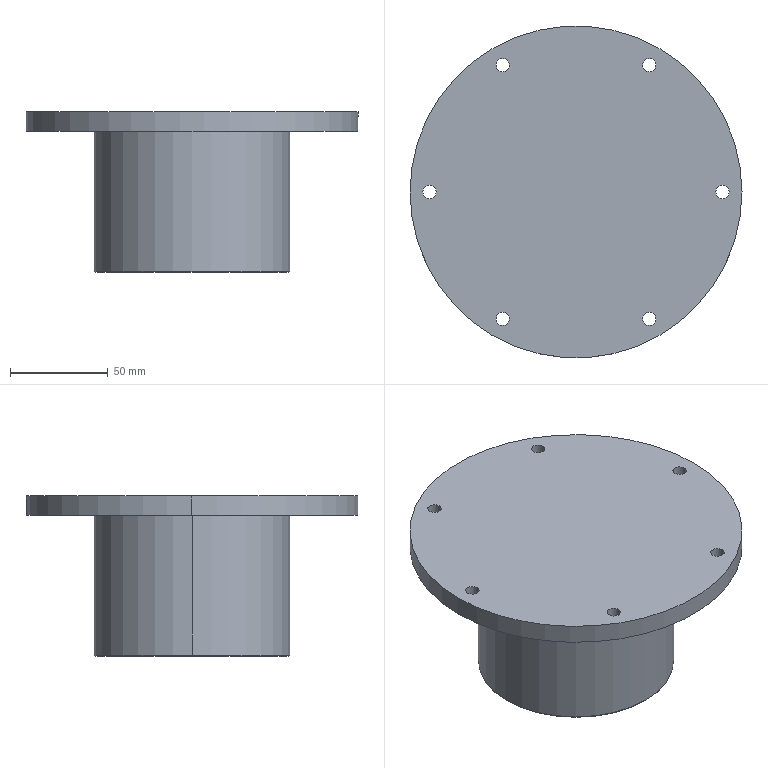Component | SolidWorks | RotatingAxis100-1 | 1 solid | 37 faces | box 170 x 170 x 82 mm | volume 789053 mm3 | cylinder 24 | cone 8 | plane 3 | torus 2 | commonest cylinder face diameters 6.8 x12 5 x8 170 x2 100 x2 | material 45#
STEP:
#1=COLOUR_RGB('',0.7922,0.8196,0.9333);
#2=FILL_AREA_STYLE_COLOUR('',#1);
#3=FILL_AREA_STYLE('',(#2));
#4=SURFACE_STYLE_FILL_AREA(#3);
#5=SURFACE_SIDE_STYLE('',(#4));
#6=SURFACE_STYLE_USAGE(.BOTH.,#5);
#7=PRESENTATION_STYLE_ASSIGNMENT((#6));
#8=CARTESIAN_POINT('',(2.019,-1.06,-50.116));
#9=VERTEX_POINT('',#8);
#10=CARTESIAN_POINT('',(-1.879,-1.06,-50.116));
#11=VERTEX_POINT('',#10);
#12=CARTESIAN_POINT('',(0.07026,-1.06,-50.116));
#13=DIRECTION('',(0.,-0.,-1.));
#14=DIRECTION('',(-1.,0.,0.));
#15=AXIS2_PLACEMENT_3D('',#12,#13,#14);
#16=CIRCLE('',#15,1.949);
#17=EDGE_CURVE('',#9,#11,#16,.T.);
#18=ORIENTED_EDGE('',*,*,#17,.F.);
#19=CARTESIAN_POINT('',(2.039,-1.06,-50.097));
#20=VERTEX_POINT('',#19);
#21=CARTESIAN_POINT('',(2.019,-1.06,-50.097));
#22=DIRECTION('',(-0.,-1.,0.));
#23=DIRECTION('',(1.,0.,0.));
#24=AXIS2_PLACEMENT_3D('',#21,#22,#23);
#25=CIRCLE('',#24,0.01969);
#26=EDGE_CURVE('',#9,#20,#25,.T.);
#27=ORIENTED_EDGE('',*,*,#26,.T.);
#28=CARTESIAN_POINT('',(-1.898,-1.06,-50.097));
#29=VERTEX_POINT('',#28);
#30=CARTESIAN_POINT('',(0.07026,-1.06,-50.097));
#31=DIRECTION('',(-0.,0.,1.));
#32=DIRECTION('',(-1.,0.,0.));
#33=AXIS2_PLACEMENT_3D('',#30,#31,#32);
#34=CIRCLE('',#33,1.969);
#35=EDGE_CURVE('',#29,#20,#34,.T.);
#36=ORIENTED_EDGE('',*,*,#35,.F.);
#37=CARTESIAN_POINT('',(-1.879,-1.06,-50.097));
#38=DIRECTION('',(0.,1.,-0.));
#39=DIRECTION('',(-1.,0.,0.));
#40=AXIS2_PLACEMENT_3D('',#37,#38,#39);
#41=CIRCLE('',#40,0.01969);
#42=EDGE_CURVE('',#11,#29,#41,.T.);
#43=ORIENTED_EDGE('',*,*,#42,.F.);
#44=EDGE_LOOP('',(#18,#27,#36,#43));
#45=FACE_OUTER_BOUND('',#44,.T.);
#46=CARTESIAN_POINT('',(0.07026,-1.06,-50.097));
#47=DIRECTION('',(-0.,0.,1.));
#48=DIRECTION('',(-1.,0.,-0.));
#49=AXIS2_PLACEMENT_3D('',#46,#47,#48);
#50=TOROIDAL_SURFACE('',#49,1.949,0.01969);
#51=ADVANCED_FACE('',(#45),#50,.T.);
#52=CARTESIAN_POINT('',(-1.142,-2.173,-49.526));
#53=VERTEX_POINT('',#52);
#54=CARTESIAN_POINT('',(-0.9449,-2.173,-49.526));
#55=VERTEX_POINT('',#54);
#56=CARTESIAN_POINT('',(-1.043,-2.173,-49.526));
#57=DIRECTION('',(0.,-0.,-1.));
#58=DIRECTION('',(1.,0.,0.));
#59=AXIS2_PLACEMENT_3D('',#56,#57,#58);
#60=CIRCLE('',#59,0.09843);
#61=EDGE_CURVE('',#53,#55,#60,.T.);
#62=ORIENTED_EDGE('',*,*,#61,.F.);
#63=CARTESIAN_POINT('',(-1.142,-2.173,-50.116));
#64=VERTEX_POINT('',#63);
#65=CARTESIAN_POINT('',(-1.142,-2.173,-50.116));
#66=DIRECTION('',(0.,-0.,-1.));
#67=VECTOR('',#66,39.37);
#68=LINE('',#65,#67);
#69=EDGE_CURVE('',#53,#64,#68,.T.);
#70=ORIENTED_EDGE('',*,*,#69,.T.);
#71=CARTESIAN_POINT('',(-0.9449,-2.173,-50.116));
#72=VERTEX_POINT('',#71);
#73=CARTESIAN_POINT('',(-1.043,-2.173,-50.116));
#74=DIRECTION('',(0.,-0.,-1.));
#75=DIRECTION('',(1.,0.,0.));
#76=AXIS2_PLACEMENT_3D('',#73,#74,#75);
#77=CIRCLE('',#76,0.09843);
#78=EDGE_CURVE('',#64,#72,#77,.T.);
#79=ORIENTED_EDGE('',*,*,#78,.T.);
#80=CARTESIAN_POINT('',(-0.9449,-2.173,-50.116));
#81=DIRECTION('',(0.,-0.,-1.));
#82=VECTOR('',#81,39.37);
#83=LINE('',#80,#82);
#84=EDGE_CURVE('',#55,#72,#83,.T.);
#85=ORIENTED_EDGE('',*,*,#84,.F.);
#86=EDGE_LOOP('',(#62,#70,#79,#85));
#87=FACE_OUTER_BOUND('',#86,.T.);
#88=CARTESIAN_POINT('',(-1.043,-2.173,-50.116));
#89=DIRECTION('',(0.,-0.,-1.));
#90=DIRECTION('',(1.,0.,0.));
#91=AXIS2_PLACEMENT_3D('',#88,#89,#90);
#92=CYLINDRICAL_SURFACE('',#91,0.09843);
#93=ADVANCED_FACE('',(#87),#92,.F.);
#94=CARTESIAN_POINT('',(-1.043,-2.173,-49.467));
#95=VERTEX_POINT('',#94);
#96=CARTESIAN_POINT('',(-0.9449,-2.173,-49.526));
#97=DIRECTION('',(0.8572,-0.,-0.515));
#98=VECTOR('',#97,39.37);
#99=LINE('',#96,#98);
#100=EDGE_CURVE('',#95,#55,#99,.T.);
#101=ORIENTED_EDGE('',*,*,#100,.F.);
#102=CARTESIAN_POINT('',(-1.142,-2.173,-49.526));
#103=DIRECTION('',(-0.8572,0.,-0.515));
#104=VECTOR('',#103,39.37);
#105=LINE('',#102,#104);
#106=EDGE_CURVE('',#95,#53,#105,.T.);
#107=ORIENTED_EDGE('',*,*,#106,.T.);
#108=ORIENTED_EDGE('',*,*,#61,.T.);
#109=EDGE_LOOP('',(#101,#107,#108));
#110=FACE_OUTER_BOUND('',#109,.T.);
#111=CARTESIAN_POINT('',(-1.043,-2.173,-49.526));
#112=DIRECTION('',(0.,-0.,-1.));
#113=DIRECTION('',(1.,0.,0.));
#114=AXIS2_PLACEMENT_3D('',#111,#112,#113);
#115=CONICAL_SURFACE('',#114,0.09843,1.03);
#116=ADVANCED_FACE('',(#110),#115,.F.);
#117=CARTESIAN_POINT('',(1.085,-2.173,-49.526));
#118=VERTEX_POINT('',#117);
#119=CARTESIAN_POINT('',(1.282,-2.173,-49.526));
#120=VERTEX_POINT('',#119);
#121=CARTESIAN_POINT('',(1.184,-2.173,-49.526));
#122=DIRECTION('',(0.,-0.,-1.));
#123=DIRECTION('',(1.,0.,0.));
#124=AXIS2_PLACEMENT_3D('',#121,#122,#123);
#125=CIRCLE('',#124,0.09843);
#126=EDGE_CURVE('',#118,#120,#125,.T.);
#127=ORIENTED_EDGE('',*,*,#126,.F.);
#128=CARTESIAN_POINT('',(1.085,-2.173,-50.116));
#129=VERTEX_POINT('',#128);
#130=CARTESIAN_POINT('',(1.085,-2.173,-50.116));
#131=DIRECTION('',(0.,-0.,-1.));
#132=VECTOR('',#131,39.37);
#133=LINE('',#130,#132);
#134=EDGE_CURVE('',#118,#129,#133,.T.);
#135=ORIENTED_EDGE('',*,*,#134,.T.);
#136=CARTESIAN_POINT('',(1.282,-2.173,-50.116));
#137=VERTEX_POINT('',#136);
#138=CARTESIAN_POINT('',(1.184,-2.173,-50.116));
#139=DIRECTION('',(0.,-0.,-1.));
#140=DIRECTION('',(1.,0.,0.));
#141=AXIS2_PLACEMENT_3D('',#138,#139,#140);
#142=CIRCLE('',#141,0.09843);
#143=EDGE_CURVE('',#129,#137,#142,.T.);
#144=ORIENTED_EDGE('',*,*,#143,.T.);
#145=CARTESIAN_POINT('',(1.282,-2.173,-50.116));
#146=DIRECTION('',(0.,-0.,-1.));
#147=VECTOR('',#146,39.37);
#148=LINE('',#145,#147);
#149=EDGE_CURVE('',#120,#137,#148,.T.);
#150=ORIENTED_EDGE('',*,*,#149,.F.);
#151=EDGE_LOOP('',(#127,#135,#144,#150));
#152=FACE_OUTER_BOUND('',#151,.T.);
#153=CARTESIAN_POINT('',(1.184,-2.173,-50.116));
#154=DIRECTION('',(0.,-0.,-1.));
#155=DIRECTION('',(1.,0.,0.));
#156=AXIS2_PLACEMENT_3D('',#153,#154,#155);
#157=CYLINDRICAL_SURFACE('',#156,0.09843);
#158=ADVANCED_FACE('',(#152),#157,.F.);
#159=CARTESIAN_POINT('',(1.184,-2.173,-49.467));
#160=VERTEX_POINT('',#159);
#161=CARTESIAN_POINT('',(1.282,-2.173,-49.526));
#162=DIRECTION('',(0.8572,-0.,-0.515));
#163=VECTOR('',#162,39.37);
#164=LINE('',#161,#163);
#165=EDGE_CURVE('',#160,#120,#164,.T.);
#166=ORIENTED_EDGE('',*,*,#165,.F.);
#167=CARTESIAN_POINT('',(1.085,-2.173,-49.526));
#168=DIRECTION('',(-0.8572,0.,-0.515));
#169=VECTOR('',#168,39.37);
#170=LINE('',#167,#169);
#171=EDGE_CURVE('',#160,#118,#170,.T.);
#172=ORIENTED_EDGE('',*,*,#171,.T.);
#173=ORIENTED_EDGE('',*,*,#126,.T.);
#174=EDGE_LOOP('',(#166,#172,#173));
#175=FACE_OUTER_BOUND('',#174,.T.);
#176=CARTESIAN_POINT('',(1.184,-2.173,-49.526));
#177=DIRECTION('',(0.,-0.,-1.));
#178=DIRECTION('',(1.,0.,0.));
#179=AXIS2_PLACEMENT_3D('',#176,#177,#178);
#180=CONICAL_SURFACE('',#179,0.09843,1.03);
#181=ADVANCED_FACE('',(#175),#180,.F.);
#182=CARTESIAN_POINT('',(1.085,0.05383,-49.526));
#183=VERTEX_POINT('',#182);
#184=CARTESIAN_POINT('',(1.282,0.05383,-49.526));
#185=VERTEX_POINT('',#184);
#186=CARTESIAN_POINT('',(1.184,0.05383,-49.526));
#187=DIRECTION('',(0.,-0.,-1.));
#188=DIRECTION('',(1.,-0.,0.));
#189=AXIS2_PLACEMENT_3D('',#186,#187,#188);
#190=CIRCLE('',#189,0.09843);
#191=EDGE_CURVE('',#183,#185,#190,.T.);
#192=ORIENTED_EDGE('',*,*,#191,.F.);
#193=CARTESIAN_POINT('',(1.085,0.05383,-50.116));
#194=VERTEX_POINT('',#193);
#195=CARTESIAN_POINT('',(1.085,0.05383,-50.116));
#196=DIRECTION('',(0.,-0.,-1.));
#197=VECTOR('',#196,39.37);
#198=LINE('',#195,#197);
#199=EDGE_CURVE('',#183,#194,#198,.T.);
#200=ORIENTED_EDGE('',*,*,#199,.T.);
#201=CARTESIAN_POINT('',(1.282,0.05383,-50.116));
#202=VERTEX_POINT('',#201);
#203=CARTESIAN_POINT('',(1.184,0.05383,-50.116));
#204=DIRECTION('',(0.,-0.,-1.));
#205=DIRECTION('',(1.,-0.,0.));
#206=AXIS2_PLACEMENT_3D('',#203,#204,#205);
#207=CIRCLE('',#206,0.09843);
#208=EDGE_CURVE('',#194,#202,#207,.T.);
#209=ORIENTED_EDGE('',*,*,#208,.T.);
#210=CARTESIAN_POINT('',(1.282,0.05383,-50.116));
#211=DIRECTION('',(0.,-0.,-1.));
#212=VECTOR('',#211,39.37);
#213=LINE('',#210,#212);
#214=EDGE_CURVE('',#185,#202,#213,.T.);
#215=ORIENTED_EDGE('',*,*,#214,.F.);
#216=EDGE_LOOP('',(#192,#200,#209,#215));
#217=FACE_OUTER_BOUND('',#216,.T.);
#218=CARTESIAN_POINT('',(1.184,0.05383,-50.116));
#219=DIRECTION('',(0.,-0.,-1.));
#220=DIRECTION('',(1.,-0.,0.));
#221=AXIS2_PLACEMENT_3D('',#218,#219,#220);
#222=CYLINDRICAL_SURFACE('',#221,0.09843);
#223=ADVANCED_FACE('',(#217),#222,.F.);
#224=CARTESIAN_POINT('',(1.184,0.05383,-49.467));
#225=VERTEX_POINT('',#224);
#226=CARTESIAN_POINT('',(1.282,0.05383,-49.526));
#227=DIRECTION('',(0.8572,-0.,-0.515));
#228=VECTOR('',#227,39.37);
#229=LINE('',#226,#228);
#230=EDGE_CURVE('',#225,#185,#229,.T.);
#231=ORIENTED_EDGE('',*,*,#230,.F.);
#232=CARTESIAN_POINT('',(1.085,0.05383,-49.526));
#233=DIRECTION('',(-0.8572,0.,-0.515));
#234=VECTOR('',#233,39.37);
#235=LINE('',#232,#234);
#236=EDGE_CURVE('',#225,#183,#235,.T.);
#237=ORIENTED_EDGE('',*,*,#236,.T.);
#238=ORIENTED_EDGE('',*,*,#191,.T.);
#239=EDGE_LOOP('',(#231,#237,#238));
#240=FACE_OUTER_BOUND('',#239,.T.);
#241=CARTESIAN_POINT('',(1.184,0.05383,-49.526));
#242=DIRECTION('',(0.,-0.,-1.));
#243=DIRECTION('',(1.,-0.,0.));
#244=AXIS2_PLACEMENT_3D('',#241,#242,#243);
#245=CONICAL_SURFACE('',#244,0.09843,1.03);
#246=ADVANCED_FACE('',(#240),#245,.F.);
#247=CARTESIAN_POINT('',(-1.142,0.05383,-49.526));
#248=VERTEX_POINT('',#247);
#249=CARTESIAN_POINT('',(-0.9449,0.05383,-49.526));
#250=VERTEX_POINT('',#249);
#251=CARTESIAN_POINT('',(-1.043,0.05383,-49.526));
#252=DIRECTION('',(0.,-0.,-1.));
#253=DIRECTION('',(1.,-0.,0.));
#254=AXIS2_PLACEMENT_3D('',#251,#252,#253);
#255=CIRCLE('',#254,0.09843);
#256=EDGE_CURVE('',#248,#250,#255,.T.);
#257=ORIENTED_EDGE('',*,*,#256,.F.);
#258=CARTESIAN_POINT('',(-1.142,0.05383,-50.116));
#259=VERTEX_POINT('',#258);
#260=CARTESIAN_POINT('',(-1.142,0.05383,-50.116));
#261=DIRECTION('',(0.,-0.,-1.));
#262=VECTOR('',#261,39.37);
#263=LINE('',#260,#262);
#264=EDGE_CURVE('',#248,#259,#263,.T.);
#265=ORIENTED_EDGE('',*,*,#264,.T.);
#266=CARTESIAN_POINT('',(-0.9449,0.05383,-50.116));
#267=VERTEX_POINT('',#266);
#268=CARTESIAN_POINT('',(-1.043,0.05383,-50.116));
#269=DIRECTION('',(0.,-0.,-1.));
#270=DIRECTION('',(1.,-0.,0.));
#271=AXIS2_PLACEMENT_3D('',#268,#269,#270);
#272=CIRCLE('',#271,0.09843);
#273=EDGE_CURVE('',#259,#267,#272,.T.);
#274=ORIENTED_EDGE('',*,*,#273,.T.);
#275=CARTESIAN_POINT('',(-0.9449,0.05383,-50.116));
#276=DIRECTION('',(0.,-0.,-1.));
#277=VECTOR('',#276,39.37);
#278=LINE('',#275,#277);
#279=EDGE_CURVE('',#250,#267,#278,.T.);
#280=ORIENTED_EDGE('',*,*,#279,.F.);
#281=EDGE_LOOP('',(#257,#265,#274,#280));
#282=FACE_OUTER_BOUND('',#281,.T.);
#283=CARTESIAN_POINT('',(-1.043,0.05383,-50.116));
#284=DIRECTION('',(0.,-0.,-1.));
#285=DIRECTION('',(1.,-0.,0.));
#286=AXIS2_PLACEMENT_3D('',#283,#284,#285);
#287=CYLINDRICAL_SURFACE('',#286,0.09843);
#288=ADVANCED_FACE('',(#282),#287,.F.);
#289=CARTESIAN_POINT('',(-1.043,0.05383,-49.467));
#290=VERTEX_POINT('',#289);
#291=CARTESIAN_POINT('',(-0.9449,0.05383,-49.526));
#292=DIRECTION('',(0.8572,-0.,-0.515));
#293=VECTOR('',#292,39.37);
#294=LINE('',#291,#293);
#295=EDGE_CURVE('',#290,#250,#294,.T.);
#296=ORIENTED_EDGE('',*,*,#295,.F.);
#297=CARTESIAN_POINT('',(-1.142,0.05383,-49.526));
#298=DIRECTION('',(-0.8572,0.,-0.515));
#299=VECTOR('',#298,39.37);
#300=LINE('',#297,#299);
#301=EDGE_CURVE('',#290,#248,#300,.T.);
#302=ORIENTED_EDGE('',*,*,#301,.T.);
#303=ORIENTED_EDGE('',*,*,#256,.T.);
#304=EDGE_LOOP('',(#296,#302,#303));
#305=FACE_OUTER_BOUND('',#304,.T.);
#306=CARTESIAN_POINT('',(-1.043,0.05383,-49.526));
#307=DIRECTION('',(0.,-0.,-1.));
#308=DIRECTION('',(1.,-0.,0.));
#309=AXIS2_PLACEMENT_3D('',#306,#307,#308);
#310=CONICAL_SURFACE('',#309,0.09843,1.03);
#311=ADVANCED_FACE('',(#305),#310,.F.);
#312=CARTESIAN_POINT('',(1.681,-3.617,-47.282));
#313=VERTEX_POINT('',#312);
#314=CARTESIAN_POINT('',(1.413,-3.617,-47.282));
#315=VERTEX_POINT('',#314);
#316=CARTESIAN_POINT('',(1.547,-3.617,-47.282));
#317=DIRECTION('',(-0.,0.,1.));
#318=DIRECTION('',(-1.,0.,0.));
#319=AXIS2_PLACEMENT_3D('',#316,#317,#318);
#320=CIRCLE('',#319,0.1339);
#321=EDGE_CURVE('',#313,#315,#320,.T.);
#322=ORIENTED_EDGE('',*,*,#321,.F.);
#323=CARTESIAN_POINT('',(1.681,-3.617,-46.888));
#324=VERTEX_POINT('',#323);
#325=CARTESIAN_POINT('',(1.681,-3.617,-46.888));
#326=DIRECTION('',(-0.,0.,1.));
#327=VECTOR('',#326,39.37);
#328=LINE('',#325,#327);
#329=EDGE_CURVE('',#313,#324,#328,.T.);
#330=ORIENTED_EDGE('',*,*,#329,.T.);
#331=CARTESIAN_POINT('',(1.413,-3.617,-46.888));
#332=VERTEX_POINT('',#331);
#333=CARTESIAN_POINT('',(1.547,-3.617,-46.888));
#334=DIRECTION('',(-0.,0.,1.));
#335=DIRECTION('',(-1.,0.,0.));
#336=AXIS2_PLACEMENT_3D('',#333,#334,#335);
#337=CIRCLE('',#336,0.1339);
#338=EDGE_CURVE('',#324,#332,#337,.T.);
#339=ORIENTED_EDGE('',*,*,#338,.T.);
#340=CARTESIAN_POINT('',(1.413,-3.617,-46.888));
#341=DIRECTION('',(-0.,0.,1.));
#342=VECTOR('',#341,39.37);
#343=LINE('',#340,#342);
#344=EDGE_CURVE('',#315,#332,#343,.T.);
#345=ORIENTED_EDGE('',*,*,#344,.F.);
#346=EDGE_LOOP('',(#322,#330,#339,#345));
#347=FACE_OUTER_BOUND('',#346,.T.);
#348=CARTESIAN_POINT('',(1.547,-3.617,-46.888));
#349=DIRECTION('',(-0.,0.,1.));
#350=DIRECTION('',(-1.,0.,0.));
#351=AXIS2_PLACEMENT_3D('',#348,#349,#350);
#352=CYLINDRICAL_SURFACE('',#351,0.1339);
#353=ADVANCED_FACE('',(#347),#352,.F.);
#354=CARTESIAN_POINT('',(-1.272,-3.617,-47.282));
#355=VERTEX_POINT('',#354);
#356=CARTESIAN_POINT('',(-1.54,-3.617,-47.282));
#357=VERTEX_POINT('',#356);
#358=CARTESIAN_POINT('',(-1.406,-3.617,-47.282));
#359=DIRECTION('',(-0.,0.,1.));
#360=DIRECTION('',(-1.,0.,0.));
#361=AXIS2_PLACEMENT_3D('',#358,#359,#360);
#362=CIRCLE('',#361,0.1339);
#363=EDGE_CURVE('',#355,#357,#362,.T.);
#364=ORIENTED_EDGE('',*,*,#363,.F.);
#365=CARTESIAN_POINT('',(-1.272,-3.617,-46.888));
#366=VERTEX_POINT('',#365);
#367=CARTESIAN_POINT('',(-1.272,-3.617,-46.888));
#368=DIRECTION('',(-0.,0.,1.));
#369=VECTOR('',#368,39.37);
#370=LINE('',#367,#369);
#371=EDGE_CURVE('',#355,#366,#370,.T.);
#372=ORIENTED_EDGE('',*,*,#371,.T.);
#373=CARTESIAN_POINT('',(-1.54,-3.617,-46.888));
#374=VERTEX_POINT('',#373);
#375=CARTESIAN_POINT('',(-1.406,-3.617,-46.888));
#376=DIRECTION('',(-0.,0.,1.));
#377=DIRECTION('',(-1.,0.,0.));
#378=AXIS2_PLACEMENT_3D('',#375,#376,#377);
#379=CIRCLE('',#378,0.1339);
#380=EDGE_CURVE('',#366,#374,#379,.T.);
#381=ORIENTED_EDGE('',*,*,#380,.T.);
#382=CARTESIAN_POINT('',(-1.54,-3.617,-46.888));
#383=DIRECTION('',(-0.,0.,1.));
#384=VECTOR('',#383,39.37);
#385=LINE('',#382,#384);
#386=EDGE_CURVE('',#357,#374,#385,.T.);
#387=ORIENTED_EDGE('',*,*,#386,.F.);
#388=EDGE_LOOP('',(#364,#372,#381,#387));
#389=FACE_OUTER_BOUND('',#388,.T.);
#390=CARTESIAN_POINT('',(-1.406,-3.617,-46.888));
#391=DIRECTION('',(-0.,0.,1.));
#392=DIRECTION('',(-1.,0.,0.));
#393=AXIS2_PLACEMENT_3D('',#390,#391,#392);
#394=CYLINDRICAL_SURFACE('',#393,0.1339);
#395=ADVANCED_FACE('',(#389),#394,.F.);
#396=CARTESIAN_POINT('',(-2.749,-1.06,-47.282));
#397=VERTEX_POINT('',#396);
#398=CARTESIAN_POINT('',(-3.016,-1.06,-47.282));
#399=VERTEX_POINT('',#398);
#400=CARTESIAN_POINT('',(-2.882,-1.06,-47.282));
#401=DIRECTION('',(-0.,0.,1.));
#402=DIRECTION('',(-1.,0.,0.));
#403=AXIS2_PLACEMENT_3D('',#400,#401,#402);
#404=CIRCLE('',#403,0.1339);
#405=EDGE_CURVE('',#397,#399,#404,.T.);
#406=ORIENTED_EDGE('',*,*,#405,.F.);
#407=CARTESIAN_POINT('',(-2.749,-1.06,-46.888));
#408=VERTEX_POINT('',#407);
#409=CARTESIAN_POINT('',(-2.749,-1.06,-46.888));
#410=DIRECTION('',(-0.,0.,1.));
#411=VECTOR('',#410,39.37);
#412=LINE('',#409,#411);
#413=EDGE_CURVE('',#397,#408,#412,.T.);
#414=ORIENTED_EDGE('',*,*,#413,.T.);
#415=CARTESIAN_POINT('',(-3.016,-1.06,-46.888));
#416=VERTEX_POINT('',#415);
#417=CARTESIAN_POINT('',(-2.882,-1.06,-46.888));
#418=DIRECTION('',(-0.,0.,1.));
#419=DIRECTION('',(-1.,0.,0.));
#420=AXIS2_PLACEMENT_3D('',#417,#418,#419);
#421=CIRCLE('',#420,0.1339);
#422=EDGE_CURVE('',#408,#416,#421,.T.);
#423=ORIENTED_EDGE('',*,*,#422,.T.);
#424=CARTESIAN_POINT('',(-3.016,-1.06,-46.888));
#425=DIRECTION('',(-0.,0.,1.));
#426=VECTOR('',#425,39.37);
#427=LINE('',#424,#426);
#428=EDGE_CURVE('',#399,#416,#427,.T.);
#429=ORIENTED_EDGE('',*,*,#428,.F.);
#430=EDGE_LOOP('',(#406,#414,#423,#429));
#431=FACE_OUTER_BOUND('',#430,.T.);
#432=CARTESIAN_POINT('',(-2.882,-1.06,-46.888));
#433=DIRECTION('',(-0.,0.,1.));
#434=DIRECTION('',(-1.,0.,0.));
#435=AXIS2_PLACEMENT_3D('',#432,#433,#434);
#436=CYLINDRICAL_SURFACE('',#435,0.1339);
#437=ADVANCED_FACE('',(#431),#436,.F.);
#438=CARTESIAN_POINT('',(-1.272,1.497,-47.282));
#439=VERTEX_POINT('',#438);
#440=CARTESIAN_POINT('',(-1.54,1.497,-47.282));
#441=VERTEX_POINT('',#440);
#442=CARTESIAN_POINT('',(-1.406,1.497,-47.282));
#443=DIRECTION('',(-0.,0.,1.));
#444=DIRECTION('',(-1.,0.,0.));
#445=AXIS2_PLACEMENT_3D('',#442,#443,#444);
#446=CIRCLE('',#445,0.1339);
#447=EDGE_CURVE('',#439,#441,#446,.T.);
#448=ORIENTED_EDGE('',*,*,#447,.F.);
#449=CARTESIAN_POINT('',(-1.272,1.497,-46.888));
#450=VERTEX_POINT('',#449);
#451=CARTESIAN_POINT('',(-1.272,1.497,-46.888));
#452=DIRECTION('',(-0.,0.,1.));
#453=VECTOR('',#452,39.37);
#454=LINE('',#451,#453);
#455=EDGE_CURVE('',#439,#450,#454,.T.);
#456=ORIENTED_EDGE('',*,*,#455,.T.);
#457=CARTESIAN_POINT('',(-1.54,1.497,-46.888));
#458=VERTEX_POINT('',#457);
#459=CARTESIAN_POINT('',(-1.406,1.497,-46.888));
#460=DIRECTION('',(-0.,0.,1.));
#461=DIRECTION('',(-1.,0.,0.));
#462=AXIS2_PLACEMENT_3D('',#459,#460,#461);
#463=CIRCLE('',#462,0.1339);
#464=EDGE_CURVE('',#450,#458,#463,.T.);
#465=ORIENTED_EDGE('',*,*,#464,.T.);
#466=CARTESIAN_POINT('',(-1.54,1.497,-46.888));
#467=DIRECTION('',(-0.,0.,1.));
#468=VECTOR('',#467,39.37);
#469=LINE('',#466,#468);
#470=EDGE_CURVE('',#441,#458,#469,.T.);
#471=ORIENTED_EDGE('',*,*,#470,.F.);
#472=EDGE_LOOP('',(#448,#456,#465,#471));
#473=FACE_OUTER_BOUND('',#472,.T.);
#474=CARTESIAN_POINT('',(-1.406,1.497,-46.888));
#475=DIRECTION('',(-0.,0.,1.));
#476=DIRECTION('',(-1.,0.,0.));
#477=AXIS2_PLACEMENT_3D('',#474,#475,#476);
#478=CYLINDRICAL_SURFACE('',#477,0.1339);
#479=ADVANCED_FACE('',(#473),#478,.F.);
#480=CARTESIAN_POINT('',(1.681,1.497,-47.282));
#481=VERTEX_POINT('',#480);
#482=CARTESIAN_POINT('',(1.413,1.497,-47.282));
#483=VERTEX_POINT('',#482);
#484=CARTESIAN_POINT('',(1.547,1.497,-47.282));
#485=DIRECTION('',(-0.,0.,1.));
#486=DIRECTION('',(-1.,0.,0.));
#487=AXIS2_PLACEMENT_3D('',#484,#485,#486);
#488=CIRCLE('',#487,0.1339);
#489=EDGE_CURVE('',#481,#483,#488,.T.);
#490=ORIENTED_EDGE('',*,*,#489,.F.);
#491=CARTESIAN_POINT('',(1.681,1.497,-46.888));
#492=VERTEX_POINT('',#491);
#493=CARTESIAN_POINT('',(1.681,1.497,-46.888));
#494=DIRECTION('',(-0.,0.,1.));
#495=VECTOR('',#494,39.37);
#496=LINE('',#493,#495);
#497=EDGE_CURVE('',#481,#492,#496,.T.);
#498=ORIENTED_EDGE('',*,*,#497,.T.);
#499=CARTESIAN_POINT('',(1.413,1.497,-46.888));
#500=VERTEX_POINT('',#499);
#501=CARTESIAN_POINT('',(1.547,1.497,-46.888));
#502=DIRECTION('',(-0.,0.,1.));
#503=DIRECTION('',(-1.,0.,0.));
#504=AXIS2_PLACEMENT_3D('',#501,#502,#503);
#505=CIRCLE('',#504,0.1339);
#506=EDGE_CURVE('',#492,#500,#505,.T.);
#507=ORIENTED_EDGE('',*,*,#506,.T.);
#508=CARTESIAN_POINT('',(1.413,1.497,-46.888));
#509=DIRECTION('',(-0.,0.,1.));
#510=VECTOR('',#509,39.37);
#511=LINE('',#508,#510);
#512=EDGE_CURVE('',#483,#500,#511,.T.);
#513=ORIENTED_EDGE('',*,*,#512,.F.);
#514=EDGE_LOOP('',(#490,#498,#507,#513));
#515=FACE_OUTER_BOUND('',#514,.T.);
#516=CARTESIAN_POINT('',(1.547,1.497,-46.888));
#517=DIRECTION('',(-0.,0.,1.));
#518=DIRECTION('',(-1.,0.,0.));
#519=AXIS2_PLACEMENT_3D('',#516,#517,#518);
#520=CYLINDRICAL_SURFACE('',#519,0.1339);
#521=ADVANCED_FACE('',(#515),#520,.F.);
#522=CARTESIAN_POINT('',(3.157,-1.06,-47.282));
#523=VERTEX_POINT('',#522);
#524=CARTESIAN_POINT('',(2.889,-1.06,-47.282));
#525=VERTEX_POINT('',#524);
#526=CARTESIAN_POINT('',(3.023,-1.06,-47.282));
#527=DIRECTION('',(-0.,0.,1.));
#528=DIRECTION('',(-1.,0.,0.));
#529=AXIS2_PLACEMENT_3D('',#526,#527,#528);
#530=CIRCLE('',#529,0.1339);
#531=EDGE_CURVE('',#523,#525,#530,.T.);
#532=ORIENTED_EDGE('',*,*,#531,.F.);
#533=CARTESIAN_POINT('',(3.157,-1.06,-46.888));
#534=VERTEX_POINT('',#533);
#535=CARTESIAN_POINT('',(3.157,-1.06,-46.888));
#536=DIRECTION('',(-0.,0.,1.));
#537=VECTOR('',#536,39.37);
#538=LINE('',#535,#537);
#539=EDGE_CURVE('',#523,#534,#538,.T.);
#540=ORIENTED_EDGE('',*,*,#539,.T.);
#541=CARTESIAN_POINT('',(2.889,-1.06,-46.888));
#542=VERTEX_POINT('',#541);
#543=CARTESIAN_POINT('',(3.023,-1.06,-46.888));
#544=DIRECTION('',(-0.,0.,1.));
#545=DIRECTION('',(-1.,0.,0.));
#546=AXIS2_PLACEMENT_3D('',#543,#544,#545);
#547=CIRCLE('',#546,0.1339);
#548=EDGE_CURVE('',#534,#542,#547,.T.);
#549=ORIENTED_EDGE('',*,*,#548,.T.);
#550=CARTESIAN_POINT('',(2.889,-1.06,-46.888));
#551=DIRECTION('',(-0.,0.,1.));
#552=VECTOR('',#551,39.37);
#553=LINE('',#550,#552);
#554=EDGE_CURVE('',#525,#542,#553,.T.);
#555=ORIENTED_EDGE('',*,*,#554,.F.);
#556=EDGE_LOOP('',(#532,#540,#549,#555));
#557=FACE_OUTER_BOUND('',#556,.T.);
#558=CARTESIAN_POINT('',(3.023,-1.06,-46.888));
#559=DIRECTION('',(-0.,0.,1.));
#560=DIRECTION('',(-1.,0.,0.));
#561=AXIS2_PLACEMENT_3D('',#558,#559,#560);
#562=CYLINDRICAL_SURFACE('',#561,0.1339);
#563=ADVANCED_FACE('',(#557),#562,.F.);
#564=CARTESIAN_POINT('',(-3.276,-1.06,-46.888));
#565=VERTEX_POINT('',#564);
#566=CARTESIAN_POINT('',(3.417,-1.06,-46.888));
#567=VERTEX_POINT('',#566);
#568=CARTESIAN_POINT('',(0.07026,-1.06,-46.888));
#569=DIRECTION('',(-0.,0.,1.));
#570=DIRECTION('',(-1.,0.,0.));
#571=AXIS2_PLACEMENT_3D('',#568,#569,#570);
#572=CIRCLE('',#571,3.346);
#573=EDGE_CURVE('',#565,#567,#572,.T.);
#574=ORIENTED_EDGE('',*,*,#573,.F.);
#575=CARTESIAN_POINT('',(-3.276,-1.06,-47.282));
#576=VERTEX_POINT('',#575);
#577=CARTESIAN_POINT('',(-3.276,-1.06,-46.888));
#578=DIRECTION('',(0.,-0.,-1.));
#579=VECTOR('',#578,39.37);
#580=LINE('',#577,#579);
#581=EDGE_CURVE('',#565,#576,#580,.T.);
#582=ORIENTED_EDGE('',*,*,#581,.T.);
#583=CARTESIAN_POINT('',(3.417,-1.06,-47.282));
#584=VERTEX_POINT('',#583);
#585=CARTESIAN_POINT('',(0.07026,-1.06,-47.282));
#586=DIRECTION('',(-0.,0.,1.));
#587=DIRECTION('',(-1.,0.,0.));
#588=AXIS2_PLACEMENT_3D('',#585,#586,#587);
#589=CIRCLE('',#588,3.346);
#590=EDGE_CURVE('',#576,#584,#589,.T.);
#591=ORIENTED_EDGE('',*,*,#590,.T.);
#592=CARTESIAN_POINT('',(3.417,-1.06,-46.888));
#593=DIRECTION('',(0.,-0.,-1.));
#594=VECTOR('',#593,39.37);
#595=LINE('',#592,#594);
#596=EDGE_CURVE('',#567,#584,#595,.T.);
#597=ORIENTED_EDGE('',*,*,#596,.F.);
#598=EDGE_LOOP('',(#574,#582,#591,#597));
#599=FACE_OUTER_BOUND('',#598,.T.);
#600=CARTESIAN_POINT('',(0.07026,-1.06,-46.888));
#601=DIRECTION('',(0.,-0.,-1.));
#602=DIRECTION('',(1.,-0.,-0.));
#603=AXIS2_PLACEMENT_3D('',#600,#601,#602);
#604=CYLINDRICAL_SURFACE('',#603,3.346);
#605=ADVANCED_FACE('',(#599),#604,.T.);
#606=CARTESIAN_POINT('',(-1.898,-1.06,-47.282));
#607=VERTEX_POINT('',#606);
#608=CARTESIAN_POINT('',(2.039,-1.06,-47.282));
#609=VERTEX_POINT('',#608);
#610=CARTESIAN_POINT('',(0.07026,-1.06,-47.282));
#611=DIRECTION('',(-0.,0.,1.));
#612=DIRECTION('',(-1.,0.,0.));
#613=AXIS2_PLACEMENT_3D('',#610,#611,#612);
#614=CIRCLE('',#613,1.969);
#615=EDGE_CURVE('',#607,#609,#614,.T.);
#616=ORIENTED_EDGE('',*,*,#615,.F.);
#617=CARTESIAN_POINT('',(-1.898,-1.06,-47.282));
#618=DIRECTION('',(0.,-0.,-1.));
#619=VECTOR('',#618,39.37);
#620=LINE('',#617,#619);
#621=EDGE_CURVE('',#607,#29,#620,.T.);
#622=ORIENTED_EDGE('',*,*,#621,.T.);
#623=ORIENTED_EDGE('',*,*,#35,.T.);
#624=CARTESIAN_POINT('',(2.039,-1.06,-47.282));
#625=DIRECTION('',(0.,-0.,-1.));
#626=VECTOR('',#625,39.37);
#627=LINE('',#624,#626);
#628=EDGE_CURVE('',#609,#20,#627,.T.);
#629=ORIENTED_EDGE('',*,*,#628,.F.);
#630=EDGE_LOOP('',(#616,#622,#623,#629));
#631=FACE_OUTER_BOUND('',#630,.T.);
#632=CARTESIAN_POINT('',(0.07026,-1.06,-47.282));
#633=DIRECTION('',(0.,-0.,-1.));
#634=DIRECTION('',(1.,-0.,0.));
#635=AXIS2_PLACEMENT_3D('',#632,#633,#634);
#636=CYLINDRICAL_SURFACE('',#635,1.969);
#637=ADVANCED_FACE('',(#631),#636,.T.);
#638=ORIENTED_EDGE('',*,*,#621,.F.);
#639=CARTESIAN_POINT('',(0.07026,-1.06,-47.282));
#640=DIRECTION('',(-0.,0.,1.));
#641=DIRECTION('',(-1.,0.,0.));
#642=AXIS2_PLACEMENT_3D('',#639,#640,#641);
#643=CIRCLE('',#642,1.969);
#644=EDGE_CURVE('',#609,#607,#643,.T.);
#645=ORIENTED_EDGE('',*,*,#644,.F.);
#646=ORIENTED_EDGE('',*,*,#628,.T.);
#647=CARTESIAN_POINT('',(0.07026,-1.06,-50.097));
#648=DIRECTION('',(-0.,0.,1.));
#649=DIRECTION('',(-1.,0.,0.));
#650=AXIS2_PLACEMENT_3D('',#647,#648,#649);
#651=CIRCLE('',#650,1.969);
#652=EDGE_CURVE('',#20,#29,#651,.T.);
#653=ORIENTED_EDGE('',*,*,#652,.T.);
#654=EDGE_LOOP('',(#638,#645,#646,#653));
#655=FACE_OUTER_BOUND('',#654,.T.);
#656=CARTESIAN_POINT('',(0.07026,-1.06,-47.282));
#657=DIRECTION('',(0.,-0.,-1.));
#658=DIRECTION('',(1.,-0.,0.));
#659=AXIS2_PLACEMENT_3D('',#656,#657,#658);
#660=CYLINDRICAL_SURFACE('',#659,1.969);
#661=ADVANCED_FACE('',(#655),#660,.T.);
#662=CARTESIAN_POINT('',(0.07026,-1.06,-50.116));
#663=DIRECTION('',(0.,-0.,-1.));
#664=DIRECTION('',(-1.,0.,0.));
#665=AXIS2_PLACEMENT_3D('',#662,#663,#664);
#666=CIRCLE('',#665,1.949);
#667=EDGE_CURVE('',#11,#9,#666,.T.);
#668=ORIENTED_EDGE('',*,*,#667,.T.);
#669=ORIENTED_EDGE('',*,*,#17,.T.);
#670=EDGE_LOOP('',(#668,#669));
#671=FACE_OUTER_BOUND('',#670,.T.);
#672=CARTESIAN_POINT('',(-1.043,-2.173,-50.116));
#673=DIRECTION('',(0.,-0.,-1.));
#674=DIRECTION('',(1.,0.,0.));
#675=AXIS2_PLACEMENT_3D('',#672,#673,#674);
#676=CIRCLE('',#675,0.09843);
#677=EDGE_CURVE('',#72,#64,#676,.T.);
#678=ORIENTED_EDGE('',*,*,#677,.F.);
#679=ORIENTED_EDGE('',*,*,#78,.F.);
#680=EDGE_LOOP('',(#678,#679));
#681=FACE_BOUND('',#680,.T.);
#682=CARTESIAN_POINT('',(1.184,-2.173,-50.116));
#683=DIRECTION('',(0.,-0.,-1.));
#684=DIRECTION('',(1.,0.,0.));
#685=AXIS2_PLACEMENT_3D('',#682,#683,#684);
#686=CIRCLE('',#685,0.09843);
#687=EDGE_CURVE('',#137,#129,#686,.T.);
#688=ORIENTED_EDGE('',*,*,#687,.F.);
#689=ORIENTED_EDGE('',*,*,#143,.F.);
#690=EDGE_LOOP('',(#688,#689));
#691=FACE_BOUND('',#690,.T.);
#692=CARTESIAN_POINT('',(1.184,0.05383,-50.116));
#693=DIRECTION('',(0.,-0.,-1.));
#694=DIRECTION('',(1.,-0.,0.));
#695=AXIS2_PLACEMENT_3D('',#692,#693,#694);
#696=CIRCLE('',#695,0.09843);
#697=EDGE_CURVE('',#202,#194,#696,.T.);
#698=ORIENTED_EDGE('',*,*,#697,.F.);
#699=ORIENTED_EDGE('',*,*,#208,.F.);
#700=EDGE_LOOP('',(#698,#699));
#701=FACE_BOUND('',#700,.T.);
#702=CARTESIAN_POINT('',(-1.043,0.05383,-50.116));
#703=DIRECTION('',(0.,-0.,-1.));
#704=DIRECTION('',(1.,-0.,0.));
#705=AXIS2_PLACEMENT_3D('',#702,#703,#704);
#706=CIRCLE('',#705,0.09843);
#707=EDGE_CURVE('',#267,#259,#706,.T.);
#708=ORIENTED_EDGE('',*,*,#707,.F.);
#709=ORIENTED_EDGE('',*,*,#273,.F.);
#710=EDGE_LOOP('',(#708,#709));
#711=FACE_BOUND('',#710,.T.);
#712=CARTESIAN_POINT('',(0.07026,-1.06,-50.116));
#713=DIRECTION('',(0.,0.,1.));
#714=DIRECTION('',(-1.,0.,0.));
#715=AXIS2_PLACEMENT_3D('',#712,#713,#714);
#716=PLANE('',#715);
#717=ADVANCED_FACE('',(#671,#681,#691,#701,#711),#716,.F.);
#718=CARTESIAN_POINT('',(1.547,-3.617,-47.282));
#719=DIRECTION('',(-0.,0.,1.));
#720=DIRECTION('',(-1.,0.,0.));
#721=AXIS2_PLACEMENT_3D('',#718,#719,#720);
#722=CIRCLE('',#721,0.1339);
#723=EDGE_CURVE('',#315,#313,#722,.T.);
#724=ORIENTED_EDGE('',*,*,#723,.T.);
#725=ORIENTED_EDGE('',*,*,#321,.T.);
#726=EDGE_LOOP('',(#724,#725));
#727=FACE_BOUND('',#726,.T.);
#728=CARTESIAN_POINT('',(-1.406,-3.617,-47.282));
#729=DIRECTION('',(-0.,0.,1.));
#730=DIRECTION('',(-1.,0.,0.));
#731=AXIS2_PLACEMENT_3D('',#728,#729,#730);
#732=CIRCLE('',#731,0.1339);
#733=EDGE_CURVE('',#357,#355,#732,.T.);
#734=ORIENTED_EDGE('',*,*,#733,.T.);
#735=ORIENTED_EDGE('',*,*,#363,.T.);
#736=EDGE_LOOP('',(#734,#735));
#737=FACE_BOUND('',#736,.T.);
#738=CARTESIAN_POINT('',(-2.882,-1.06,-47.282));
#739=DIRECTION('',(-0.,0.,1.));
#740=DIRECTION('',(-1.,0.,0.));
#741=AXIS2_PLACEMENT_3D('',#738,#739,#740);
#742=CIRCLE('',#741,0.1339);
#743=EDGE_CURVE('',#399,#397,#742,.T.);
#744=ORIENTED_EDGE('',*,*,#743,.T.);
#745=ORIENTED_EDGE('',*,*,#405,.T.);
#746=EDGE_LOOP('',(#744,#745));
#747=FACE_BOUND('',#746,.T.);
#748=CARTESIAN_POINT('',(-1.406,1.497,-47.282));
#749=DIRECTION('',(-0.,0.,1.));
#750=DIRECTION('',(-1.,0.,0.));
#751=AXIS2_PLACEMENT_3D('',#748,#749,#750);
#752=CIRCLE('',#751,0.1339);
#753=EDGE_CURVE('',#441,#439,#752,.T.);
#754=ORIENTED_EDGE('',*,*,#753,.T.);
#755=ORIENTED_EDGE('',*,*,#447,.T.);
#756=EDGE_LOOP('',(#754,#755));
#757=FACE_BOUND('',#756,.T.);
#758=CARTESIAN_POINT('',(1.547,1.497,-47.282));
#759=DIRECTION('',(-0.,0.,1.));
#760=DIRECTION('',(-1.,0.,0.));
#761=AXIS2_PLACEMENT_3D('',#758,#759,#760);
#762=CIRCLE('',#761,0.1339);
#763=EDGE_CURVE('',#483,#481,#762,.T.);
#764=ORIENTED_EDGE('',*,*,#763,.T.);
#765=ORIENTED_EDGE('',*,*,#489,.T.);
#766=EDGE_LOOP('',(#764,#765));
#767=FACE_BOUND('',#766,.T.);
#768=CARTESIAN_POINT('',(3.023,-1.06,-47.282));
#769=DIRECTION('',(-0.,0.,1.));
#770=DIRECTION('',(-1.,0.,0.));
#771=AXIS2_PLACEMENT_3D('',#768,#769,#770);
#772=CIRCLE('',#771,0.1339);
#773=EDGE_CURVE('',#525,#523,#772,.T.);
#774=ORIENTED_EDGE('',*,*,#773,.T.);
#775=ORIENTED_EDGE('',*,*,#531,.T.);
#776=EDGE_LOOP('',(#774,#775));
#777=FACE_BOUND('',#776,.T.);
#778=CARTESIAN_POINT('',(0.07026,-1.06,-47.282));
#779=DIRECTION('',(-0.,0.,1.));
#780=DIRECTION('',(-1.,0.,0.));
#781=AXIS2_PLACEMENT_3D('',#778,#779,#780);
#782=CIRCLE('',#781,3.346);
#783=EDGE_CURVE('',#584,#576,#782,.T.);
#784=ORIENTED_EDGE('',*,*,#783,.F.);
#785=ORIENTED_EDGE('',*,*,#590,.F.);
#786=EDGE_LOOP('',(#784,#785));
#787=FACE_OUTER_BOUND('',#786,.T.);
#788=ORIENTED_EDGE('',*,*,#644,.T.);
#789=ORIENTED_EDGE('',*,*,#615,.T.);
#790=EDGE_LOOP('',(#788,#789));
#791=FACE_BOUND('',#790,.T.);
#792=CARTESIAN_POINT('',(0.07026,-1.06,-47.282));
#793=DIRECTION('',(0.,0.,1.));
#794=DIRECTION('',(-1.,0.,0.));
#795=AXIS2_PLACEMENT_3D('',#792,#793,#794);
#796=PLANE('',#795);
#797=ADVANCED_FACE('',(#727,#737,#747,#757,#767,#777,#787,#791),#796,.F.);
#798=ORIENTED_EDGE('',*,*,#581,.F.);
#799=CARTESIAN_POINT('',(0.07026,-1.06,-46.888));
#800=DIRECTION('',(-0.,0.,1.));
#801=DIRECTION('',(-1.,0.,0.));
#802=AXIS2_PLACEMENT_3D('',#799,#800,#801);
#803=CIRCLE('',#802,3.346);
#804=EDGE_CURVE('',#567,#565,#803,.T.);
#805=ORIENTED_EDGE('',*,*,#804,.F.);
#806=ORIENTED_EDGE('',*,*,#596,.T.);
#807=ORIENTED_EDGE('',*,*,#783,.T.);
#808=EDGE_LOOP('',(#798,#805,#806,#807));
#809=FACE_OUTER_BOUND('',#808,.T.);
#810=CARTESIAN_POINT('',(0.07026,-1.06,-46.888));
#811=DIRECTION('',(0.,-0.,-1.));
#812=DIRECTION('',(1.,-0.,-0.));
#813=AXIS2_PLACEMENT_3D('',#810,#811,#812);
#814=CYLINDRICAL_SURFACE('',#813,3.346);
#815=ADVANCED_FACE('',(#809),#814,.T.);
#816=CARTESIAN_POINT('',(1.547,-3.617,-46.888));
#817=DIRECTION('',(-0.,0.,1.));
#818=DIRECTION('',(-1.,0.,0.));
#819=AXIS2_PLACEMENT_3D('',#816,#817,#818);
#820=CIRCLE('',#819,0.1339);
#821=EDGE_CURVE('',#332,#324,#820,.T.);
#822=ORIENTED_EDGE('',*,*,#821,.F.);
#823=ORIENTED_EDGE('',*,*,#338,.F.);
#824=EDGE_LOOP('',(#822,#823));
#825=FACE_BOUND('',#824,.T.);
#826=CARTESIAN_POINT('',(-1.406,-3.617,-46.888));
#827=DIRECTION('',(-0.,0.,1.));
#828=DIRECTION('',(-1.,0.,0.));
#829=AXIS2_PLACEMENT_3D('',#826,#827,#828);
#830=CIRCLE('',#829,0.1339);
#831=EDGE_CURVE('',#374,#366,#830,.T.);
#832=ORIENTED_EDGE('',*,*,#831,.F.);
#833=ORIENTED_EDGE('',*,*,#380,.F.);
#834=EDGE_LOOP('',(#832,#833));
#835=FACE_BOUND('',#834,.T.);
#836=CARTESIAN_POINT('',(-2.882,-1.06,-46.888));
#837=DIRECTION('',(-0.,0.,1.));
#838=DIRECTION('',(-1.,0.,0.));
#839=AXIS2_PLACEMENT_3D('',#836,#837,#838);
#840=CIRCLE('',#839,0.1339);
#841=EDGE_CURVE('',#416,#408,#840,.T.);
#842=ORIENTED_EDGE('',*,*,#841,.F.);
#843=ORIENTED_EDGE('',*,*,#422,.F.);
#844=EDGE_LOOP('',(#842,#843));
#845=FACE_BOUND('',#844,.T.);
#846=CARTESIAN_POINT('',(-1.406,1.497,-46.888));
#847=DIRECTION('',(-0.,0.,1.));
#848=DIRECTION('',(-1.,0.,0.));
#849=AXIS2_PLACEMENT_3D('',#846,#847,#848);
#850=CIRCLE('',#849,0.1339);
#851=EDGE_CURVE('',#458,#450,#850,.T.);
#852=ORIENTED_EDGE('',*,*,#851,.F.);
#853=ORIENTED_EDGE('',*,*,#464,.F.);
#854=EDGE_LOOP('',(#852,#853));
#855=FACE_BOUND('',#854,.T.);
#856=CARTESIAN_POINT('',(1.547,1.497,-46.888));
#857=DIRECTION('',(-0.,0.,1.));
#858=DIRECTION('',(-1.,0.,0.));
#859=AXIS2_PLACEMENT_3D('',#856,#857,#858);
#860=CIRCLE('',#859,0.1339);
#861=EDGE_CURVE('',#500,#492,#860,.T.);
#862=ORIENTED_EDGE('',*,*,#861,.F.);
#863=ORIENTED_EDGE('',*,*,#506,.F.);
#864=EDGE_LOOP('',(#862,#863));
#865=FACE_BOUND('',#864,.T.);
#866=CARTESIAN_POINT('',(3.023,-1.06,-46.888));
#867=DIRECTION('',(-0.,0.,1.));
#868=DIRECTION('',(-1.,0.,0.));
#869=AXIS2_PLACEMENT_3D('',#866,#867,#868);
#870=CIRCLE('',#869,0.1339);
#871=EDGE_CURVE('',#542,#534,#870,.T.);
#872=ORIENTED_EDGE('',*,*,#871,.F.);
#873=ORIENTED_EDGE('',*,*,#548,.F.);
#874=EDGE_LOOP('',(#872,#873));
#875=FACE_BOUND('',#874,.T.);
#876=ORIENTED_EDGE('',*,*,#804,.T.);
#877=ORIENTED_EDGE('',*,*,#573,.T.);
#878=EDGE_LOOP('',(#876,#877));
#879=FACE_OUTER_BOUND('',#878,.T.);
#880=CARTESIAN_POINT('',(0.07026,-1.06,-46.888));
#881=DIRECTION('',(0.,0.,1.));
#882=DIRECTION('',(-1.,0.,0.));
#883=AXIS2_PLACEMENT_3D('',#880,#881,#882);
#884=PLANE('',#883);
#885=ADVANCED_FACE('',(#825,#835,#845,#855,#865,#875,#879),#884,.T.);
#886=ORIENTED_EDGE('',*,*,#539,.F.);
#887=ORIENTED_EDGE('',*,*,#773,.F.);
#888=ORIENTED_EDGE('',*,*,#554,.T.);
#889=ORIENTED_EDGE('',*,*,#871,.T.);
#890=EDGE_LOOP('',(#886,#887,#888,#889));
#891=FACE_OUTER_BOUND('',#890,.T.);
#892=CARTESIAN_POINT('',(3.023,-1.06,-46.888));
#893=DIRECTION('',(-0.,0.,1.));
#894=DIRECTION('',(-1.,0.,0.));
#895=AXIS2_PLACEMENT_3D('',#892,#893,#894);
#896=CYLINDRICAL_SURFACE('',#895,0.1339);
#897=ADVANCED_FACE('',(#891),#896,.F.);
#898=ORIENTED_EDGE('',*,*,#497,.F.);
#899=ORIENTED_EDGE('',*,*,#763,.F.);
#900=ORIENTED_EDGE('',*,*,#512,.T.);
#901=ORIENTED_EDGE('',*,*,#861,.T.);
#902=EDGE_LOOP('',(#898,#899,#900,#901));
#903=FACE_OUTER_BOUND('',#902,.T.);
#904=CARTESIAN_POINT('',(1.547,1.497,-46.888));
#905=DIRECTION('',(-0.,0.,1.));
#906=DIRECTION('',(-1.,0.,0.));
#907=AXIS2_PLACEMENT_3D('',#904,#905,#906);
#908=CYLINDRICAL_SURFACE('',#907,0.1339);
#909=ADVANCED_FACE('',(#903),#908,.F.);
#910=ORIENTED_EDGE('',*,*,#455,.F.);
#911=ORIENTED_EDGE('',*,*,#753,.F.);
#912=ORIENTED_EDGE('',*,*,#470,.T.);
#913=ORIENTED_EDGE('',*,*,#851,.T.);
#914=EDGE_LOOP('',(#910,#911,#912,#913));
#915=FACE_OUTER_BOUND('',#914,.T.);
#916=CARTESIAN_POINT('',(-1.406,1.497,-46.888));
#917=DIRECTION('',(-0.,0.,1.));
#918=DIRECTION('',(-1.,0.,0.));
#919=AXIS2_PLACEMENT_3D('',#916,#917,#918);
#920=CYLINDRICAL_SURFACE('',#919,0.1339);
#921=ADVANCED_FACE('',(#915),#920,.F.);
#922=ORIENTED_EDGE('',*,*,#413,.F.);
#923=ORIENTED_EDGE('',*,*,#743,.F.);
#924=ORIENTED_EDGE('',*,*,#428,.T.);
#925=ORIENTED_EDGE('',*,*,#841,.T.);
#926=EDGE_LOOP('',(#922,#923,#924,#925));
#927=FACE_OUTER_BOUND('',#926,.T.);
#928=CARTESIAN_POINT('',(-2.882,-1.06,-46.888));
#929=DIRECTION('',(-0.,0.,1.));
#930=DIRECTION('',(-1.,0.,0.));
#931=AXIS2_PLACEMENT_3D('',#928,#929,#930);
#932=CYLINDRICAL_SURFACE('',#931,0.1339);
#933=ADVANCED_FACE('',(#927),#932,.F.);
#934=ORIENTED_EDGE('',*,*,#371,.F.);
#935=ORIENTED_EDGE('',*,*,#733,.F.);
#936=ORIENTED_EDGE('',*,*,#386,.T.);
#937=ORIENTED_EDGE('',*,*,#831,.T.);
#938=EDGE_LOOP('',(#934,#935,#936,#937));
#939=FACE_OUTER_BOUND('',#938,.T.);
#940=CARTESIAN_POINT('',(-1.406,-3.617,-46.888));
#941=DIRECTION('',(-0.,0.,1.));
#942=DIRECTION('',(-1.,0.,0.));
#943=AXIS2_PLACEMENT_3D('',#940,#941,#942);
#944=CYLINDRICAL_SURFACE('',#943,0.1339);
#945=ADVANCED_FACE('',(#939),#944,.F.);
#946=ORIENTED_EDGE('',*,*,#329,.F.);
#947=ORIENTED_EDGE('',*,*,#723,.F.);
#948=ORIENTED_EDGE('',*,*,#344,.T.);
#949=ORIENTED_EDGE('',*,*,#821,.T.);
#950=EDGE_LOOP('',(#946,#947,#948,#949));
#951=FACE_OUTER_BOUND('',#950,.T.);
#952=CARTESIAN_POINT('',(1.547,-3.617,-46.888));
#953=DIRECTION('',(-0.,0.,1.));
#954=DIRECTION('',(-1.,0.,0.));
#955=AXIS2_PLACEMENT_3D('',#952,#953,#954);
#956=CYLINDRICAL_SURFACE('',#955,0.1339);
#957=ADVANCED_FACE('',(#951),#956,.F.);
#958=ORIENTED_EDGE('',*,*,#301,.F.);
#959=ORIENTED_EDGE('',*,*,#295,.T.);
#960=CARTESIAN_POINT('',(-1.043,0.05383,-49.526));
#961=DIRECTION('',(0.,-0.,-1.));
#962=DIRECTION('',(1.,-0.,0.));
#963=AXIS2_PLACEMENT_3D('',#960,#961,#962);
#964=CIRCLE('',#963,0.09843);
#965=EDGE_CURVE('',#250,#248,#964,.T.);
#966=ORIENTED_EDGE('',*,*,#965,.T.);
#967=EDGE_LOOP('',(#958,#959,#966));
#968=FACE_OUTER_BOUND('',#967,.T.);
#969=CARTESIAN_POINT('',(-1.043,0.05383,-49.526));
#970=DIRECTION('',(0.,-0.,-1.));
#971=DIRECTION('',(1.,-0.,0.));
#972=AXIS2_PLACEMENT_3D('',#969,#970,#971);
#973=CONICAL_SURFACE('',#972,0.09843,1.03);
#974=ADVANCED_FACE('',(#968),#973,.F.);
#975=ORIENTED_EDGE('',*,*,#264,.F.);
#976=ORIENTED_EDGE('',*,*,#965,.F.);
#977=ORIENTED_EDGE('',*,*,#279,.T.);
#978=ORIENTED_EDGE('',*,*,#707,.T.);
#979=EDGE_LOOP('',(#975,#976,#977,#978));
#980=FACE_OUTER_BOUND('',#979,.T.);
#981=CARTESIAN_POINT('',(-1.043,0.05383,-50.116));
#982=DIRECTION('',(0.,-0.,-1.));
#983=DIRECTION('',(1.,-0.,0.));
#984=AXIS2_PLACEMENT_3D('',#981,#982,#983);
#985=CYLINDRICAL_SURFACE('',#984,0.09843);
#986=ADVANCED_FACE('',(#980),#985,.F.);
#987=ORIENTED_EDGE('',*,*,#236,.F.);
#988=ORIENTED_EDGE('',*,*,#230,.T.);
#989=CARTESIAN_POINT('',(1.184,0.05383,-49.526));
#990=DIRECTION('',(0.,-0.,-1.));
#991=DIRECTION('',(1.,-0.,0.));
#992=AXIS2_PLACEMENT_3D('',#989,#990,#991);
#993=CIRCLE('',#992,0.09843);
#994=EDGE_CURVE('',#185,#183,#993,.T.);
#995=ORIENTED_EDGE('',*,*,#994,.T.);
#996=EDGE_LOOP('',(#987,#988,#995));
#997=FACE_OUTER_BOUND('',#996,.T.);
#998=CARTESIAN_POINT('',(1.184,0.05383,-49.526));
#999=DIRECTION('',(0.,-0.,-1.));
#1000=DIRECTION('',(1.,-0.,0.));
#1001=AXIS2_PLACEMENT_3D('',#998,#999,#1000);
#1002=CONICAL_SURFACE('',#1001,0.09843,1.03);
#1003=ADVANCED_FACE('',(#997),#1002,.F.);
#1004=ORIENTED_EDGE('',*,*,#199,.F.);
#1005=ORIENTED_EDGE('',*,*,#994,.F.);
#1006=ORIENTED_EDGE('',*,*,#214,.T.);
#1007=ORIENTED_EDGE('',*,*,#697,.T.);
#1008=EDGE_LOOP('',(#1004,#1005,#1006,#1007));
#1009=FACE_OUTER_BOUND('',#1008,.T.);
#1010=CARTESIAN_POINT('',(1.184,0.05383,-50.116));
#1011=DIRECTION('',(0.,-0.,-1.));
#1012=DIRECTION('',(1.,-0.,0.));
#1013=AXIS2_PLACEMENT_3D('',#1010,#1011,#1012);
#1014=CYLINDRICAL_SURFACE('',#1013,0.09843);
#1015=ADVANCED_FACE('',(#1009),#1014,.F.);
#1016=ORIENTED_EDGE('',*,*,#171,.F.);
#1017=ORIENTED_EDGE('',*,*,#165,.T.);
#1018=CARTESIAN_POINT('',(1.184,-2.173,-49.526));
#1019=DIRECTION('',(0.,-0.,-1.));
#1020=DIRECTION('',(1.,0.,0.));
#1021=AXIS2_PLACEMENT_3D('',#1018,#1019,#1020);
#1022=CIRCLE('',#1021,0.09843);
#1023=EDGE_CURVE('',#120,#118,#1022,.T.);
#1024=ORIENTED_EDGE('',*,*,#1023,.T.);
#1025=EDGE_LOOP('',(#1016,#1017,#1024));
#1026=FACE_OUTER_BOUND('',#1025,.T.);
#1027=CARTESIAN_POINT('',(1.184,-2.173,-49.526));
#1028=DIRECTION('',(0.,-0.,-1.));
#1029=DIRECTION('',(1.,0.,0.));
#1030=AXIS2_PLACEMENT_3D('',#1027,#1028,#1029);
#1031=CONICAL_SURFACE('',#1030,0.09843,1.03);
#1032=ADVANCED_FACE('',(#1026),#1031,.F.);
#1033=ORIENTED_EDGE('',*,*,#134,.F.);
#1034=ORIENTED_EDGE('',*,*,#1023,.F.);
#1035=ORIENTED_EDGE('',*,*,#149,.T.);
#1036=ORIENTED_EDGE('',*,*,#687,.T.);
#1037=EDGE_LOOP('',(#1033,#1034,#1035,#1036));
#1038=FACE_OUTER_BOUND('',#1037,.T.);
#1039=CARTESIAN_POINT('',(1.184,-2.173,-50.116));
#1040=DIRECTION('',(0.,-0.,-1.));
#1041=DIRECTION('',(1.,0.,0.));
#1042=AXIS2_PLACEMENT_3D('',#1039,#1040,#1041);
#1043=CYLINDRICAL_SURFACE('',#1042,0.09843);
#1044=ADVANCED_FACE('',(#1038),#1043,.F.);
#1045=ORIENTED_EDGE('',*,*,#106,.F.);
#1046=ORIENTED_EDGE('',*,*,#100,.T.);
#1047=CARTESIAN_POINT('',(-1.043,-2.173,-49.526));
#1048=DIRECTION('',(0.,-0.,-1.));
#1049=DIRECTION('',(1.,0.,0.));
#1050=AXIS2_PLACEMENT_3D('',#1047,#1048,#1049);
#1051=CIRCLE('',#1050,0.09843);
#1052=EDGE_CURVE('',#55,#53,#1051,.T.);
#1053=ORIENTED_EDGE('',*,*,#1052,.T.);
#1054=EDGE_LOOP('',(#1045,#1046,#1053));
#1055=FACE_OUTER_BOUND('',#1054,.T.);
#1056=CARTESIAN_POINT('',(-1.043,-2.173,-49.526));
#1057=DIRECTION('',(0.,-0.,-1.));
#1058=DIRECTION('',(1.,0.,0.));
#1059=AXIS2_PLACEMENT_3D('',#1056,#1057,#1058);
#1060=CONICAL_SURFACE('',#1059,0.09843,1.03);
#1061=ADVANCED_FACE('',(#1055),#1060,.F.);
#1062=ORIENTED_EDGE('',*,*,#69,.F.);
#1063=ORIENTED_EDGE('',*,*,#1052,.F.);
#1064=ORIENTED_EDGE('',*,*,#84,.T.);
#1065=ORIENTED_EDGE('',*,*,#677,.T.);
#1066=EDGE_LOOP('',(#1062,#1063,#1064,#1065));
#1067=FACE_OUTER_BOUND('',#1066,.T.);
#1068=CARTESIAN_POINT('',(-1.043,-2.173,-50.116));
#1069=DIRECTION('',(0.,-0.,-1.));
#1070=DIRECTION('',(1.,0.,0.));
#1071=AXIS2_PLACEMENT_3D('',#1068,#1069,#1070);
#1072=CYLINDRICAL_SURFACE('',#1071,0.09843);
#1073=ADVANCED_FACE('',(#1067),#1072,.F.);
#1074=ORIENTED_EDGE('',*,*,#26,.F.);
#1075=ORIENTED_EDGE('',*,*,#667,.F.);
#1076=ORIENTED_EDGE('',*,*,#42,.T.);
#1077=ORIENTED_EDGE('',*,*,#652,.F.);
#1078=EDGE_LOOP('',(#1074,#1075,#1076,#1077));
#1079=FACE_OUTER_BOUND('',#1078,.T.);
#1080=CARTESIAN_POINT('',(0.07026,-1.06,-50.097));
#1081=DIRECTION('',(-0.,0.,1.));
#1082=DIRECTION('',(-1.,0.,-0.));
#1083=AXIS2_PLACEMENT_3D('',#1080,#1081,#1082);
#1084=TOROIDAL_SURFACE('',#1083,1.949,0.01969);
#1085=ADVANCED_FACE('',(#1079),#1084,.T.);
#1086=CLOSED_SHELL('',(#51,#93,#116,#158,#181,#223,#246,#288,#311,#353,#395,#437,#479,#521,#563,#605,#637,#661,#717,#797,#815,#885,#897,#909,#921,#933,#945,#957,#974,#986,#1003,#1015,#1032,#1044,#1061,#1073,#1085));
#1087=MANIFOLD_SOLID_BREP('',#1086);
#1088=STYLED_ITEM('',(#7),#1087);
#1089=PRESENTATION_LAYER_ASSIGNMENT('','',(#1088));
#1090=CARTESIAN_POINT('',(0.,0.,0.));
#1091=DIRECTION('',(0.,0.,1.));
#1092=DIRECTION('',(1.,0.,0.));
#1093=AXIS2_PLACEMENT_3D('',#1090,#1091,#1092);
#1094=(LENGTH_UNIT()NAMED_UNIT(*)SI_UNIT($,.METRE.));
#1095=LENGTH_MEASURE_WITH_UNIT(LENGTH_MEASURE(0.0254),#1094);
#1096=DIMENSIONAL_EXPONENTS(1.,0.,0.,0.,0.,0.,0.);
#1097=(CONVERSION_BASED_UNIT('',#1095)LENGTH_UNIT()NAMED_UNIT(#1096));
#1098=UNCERTAINTY_MEASURE_WITH_UNIT(LENGTH_MEASURE(0.00001),#1097,'','');
#1099=(NAMED_UNIT(*)PLANE_ANGLE_UNIT()SI_UNIT($,.RADIAN.));
#1100=(NAMED_UNIT(*)SI_UNIT($,.STERADIAN.)SOLID_ANGLE_UNIT());
#1101=(GEOMETRIC_REPRESENTATION_CONTEXT(3)GLOBAL_UNCERTAINTY_ASSIGNED_CONTEXT((#1098))GLOBAL_UNIT_ASSIGNED_CONTEXT((#1097,#1099,#1100))REPRESENTATION_CONTEXT('',''));
#1102=ADVANCED_BREP_SHAPE_REPRESENTATION('',(#1087,#1093),#1101);
#1103=(LENGTH_UNIT()NAMED_UNIT(*)SI_UNIT($,.METRE.));
#1104=LENGTH_MEASURE_WITH_UNIT(LENGTH_MEASURE(0.0254),#1103);
#1105=DIMENSIONAL_EXPONENTS(1.,0.,0.,0.,0.,0.,0.);
#1106=(CONVERSION_BASED_UNIT('',#1104)LENGTH_UNIT()NAMED_UNIT(#1105));
#1107=UNCERTAINTY_MEASURE_WITH_UNIT(LENGTH_MEASURE(0.00001),#1106,'','');
#1108=(NAMED_UNIT(*)PLANE_ANGLE_UNIT()SI_UNIT($,.RADIAN.));
#1109=(NAMED_UNIT(*)SI_UNIT($,.STERADIAN.)SOLID_ANGLE_UNIT());
#1110=(GEOMETRIC_REPRESENTATION_CONTEXT(3)GLOBAL_UNCERTAINTY_ASSIGNED_CONTEXT((#1107))GLOBAL_UNIT_ASSIGNED_CONTEXT((#1106,#1108,#1109))REPRESENTATION_CONTEXT('',''));
#1111=MECHANICAL_DESIGN_GEOMETRIC_PRESENTATION_REPRESENTATION('',(#1088),#1110);